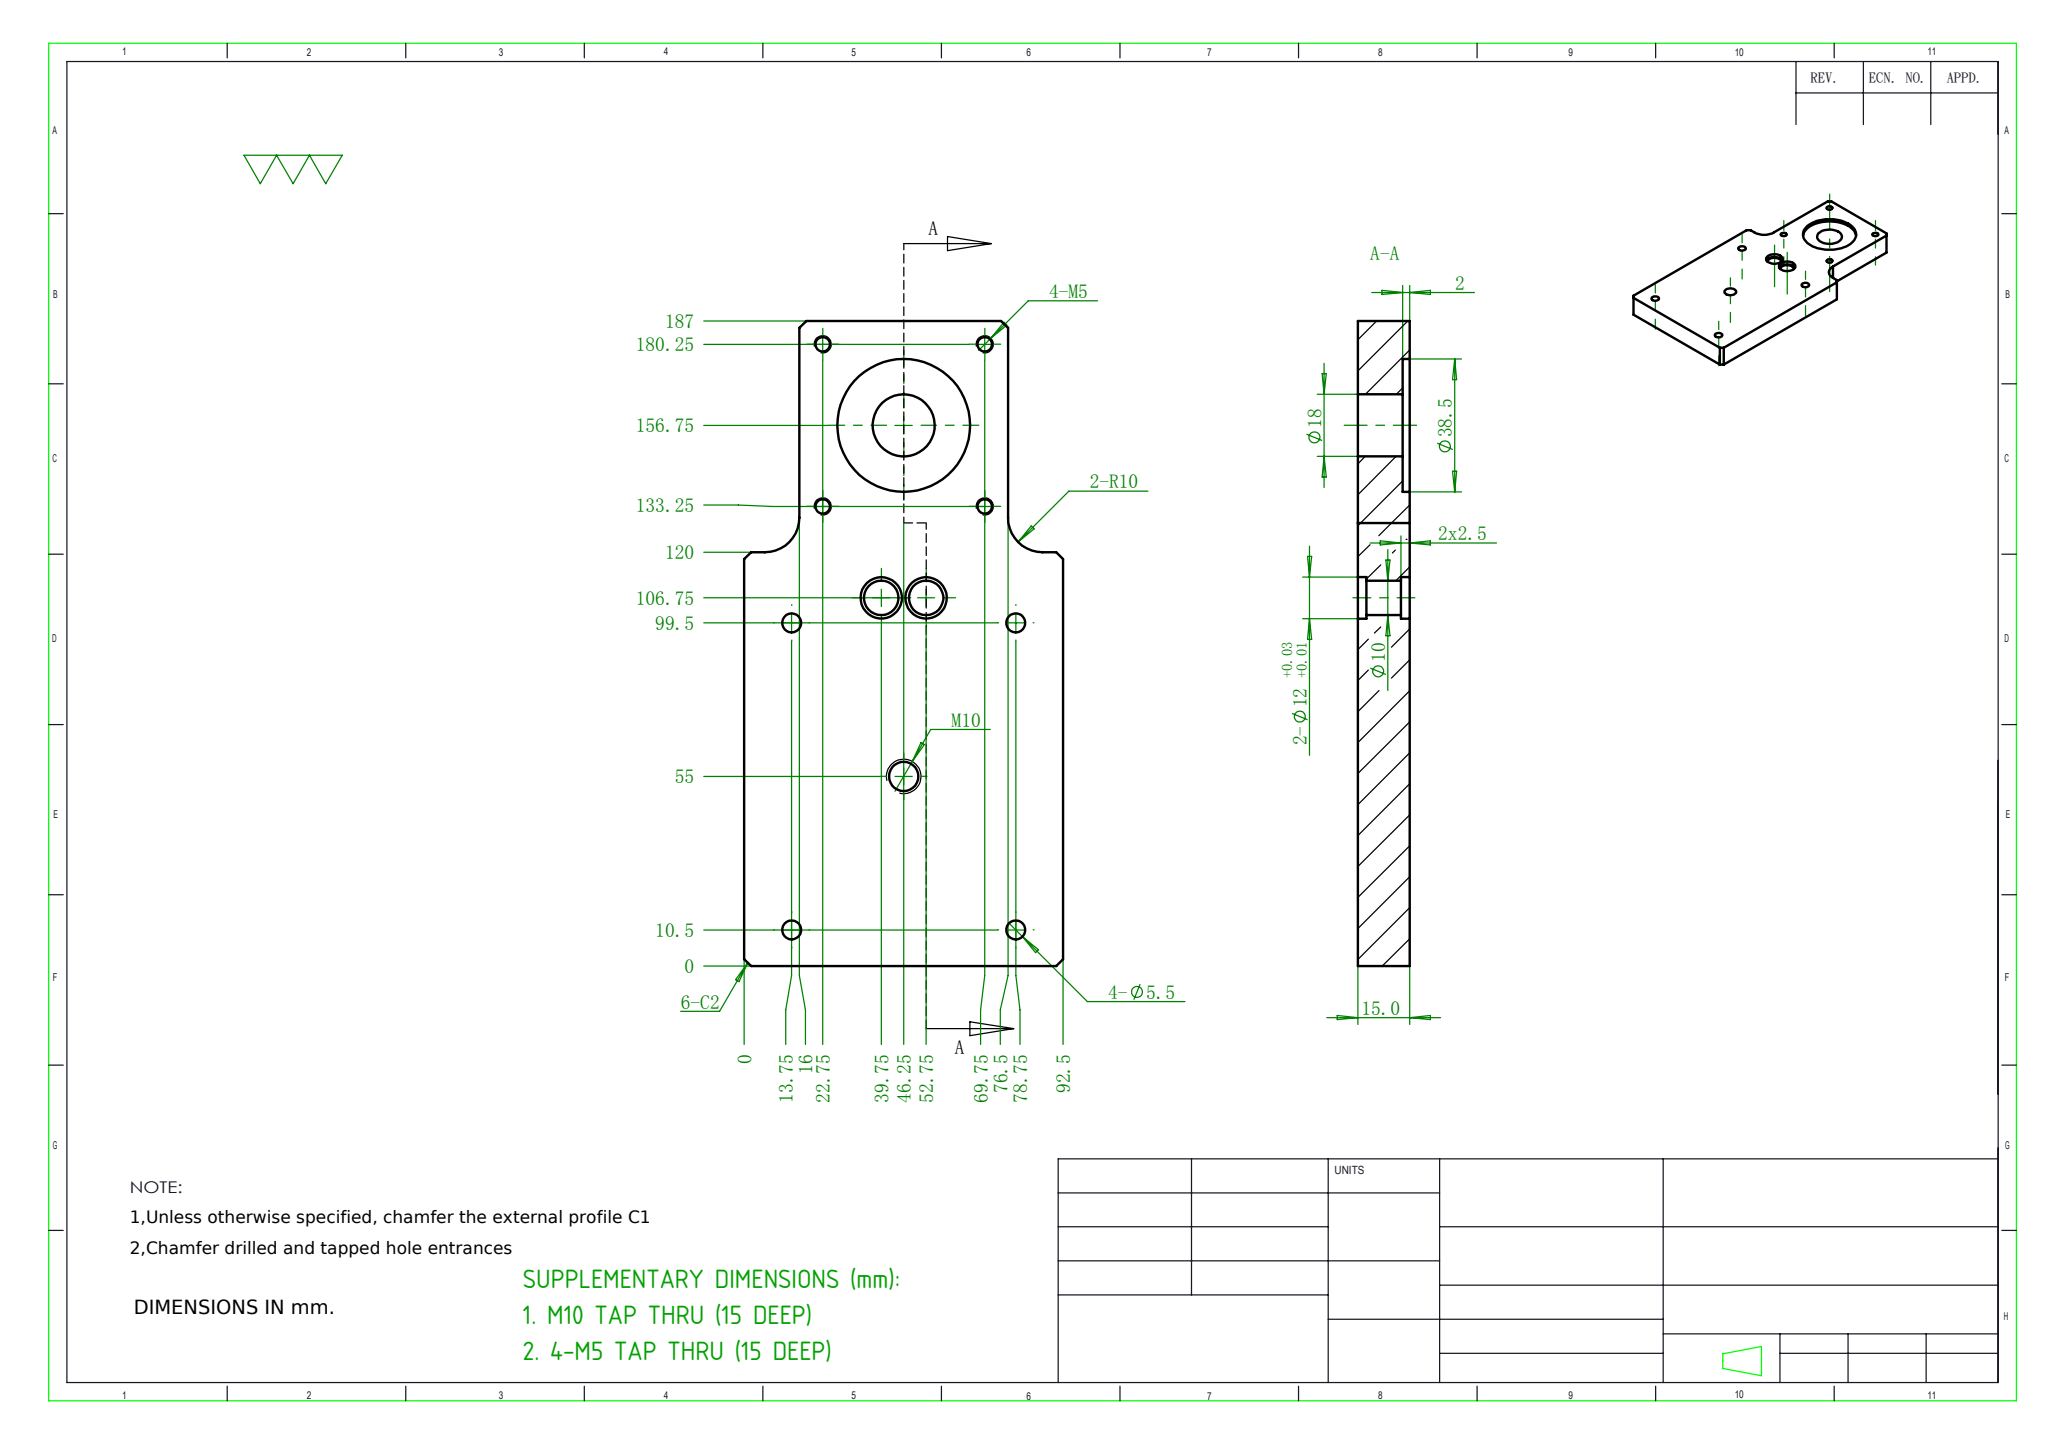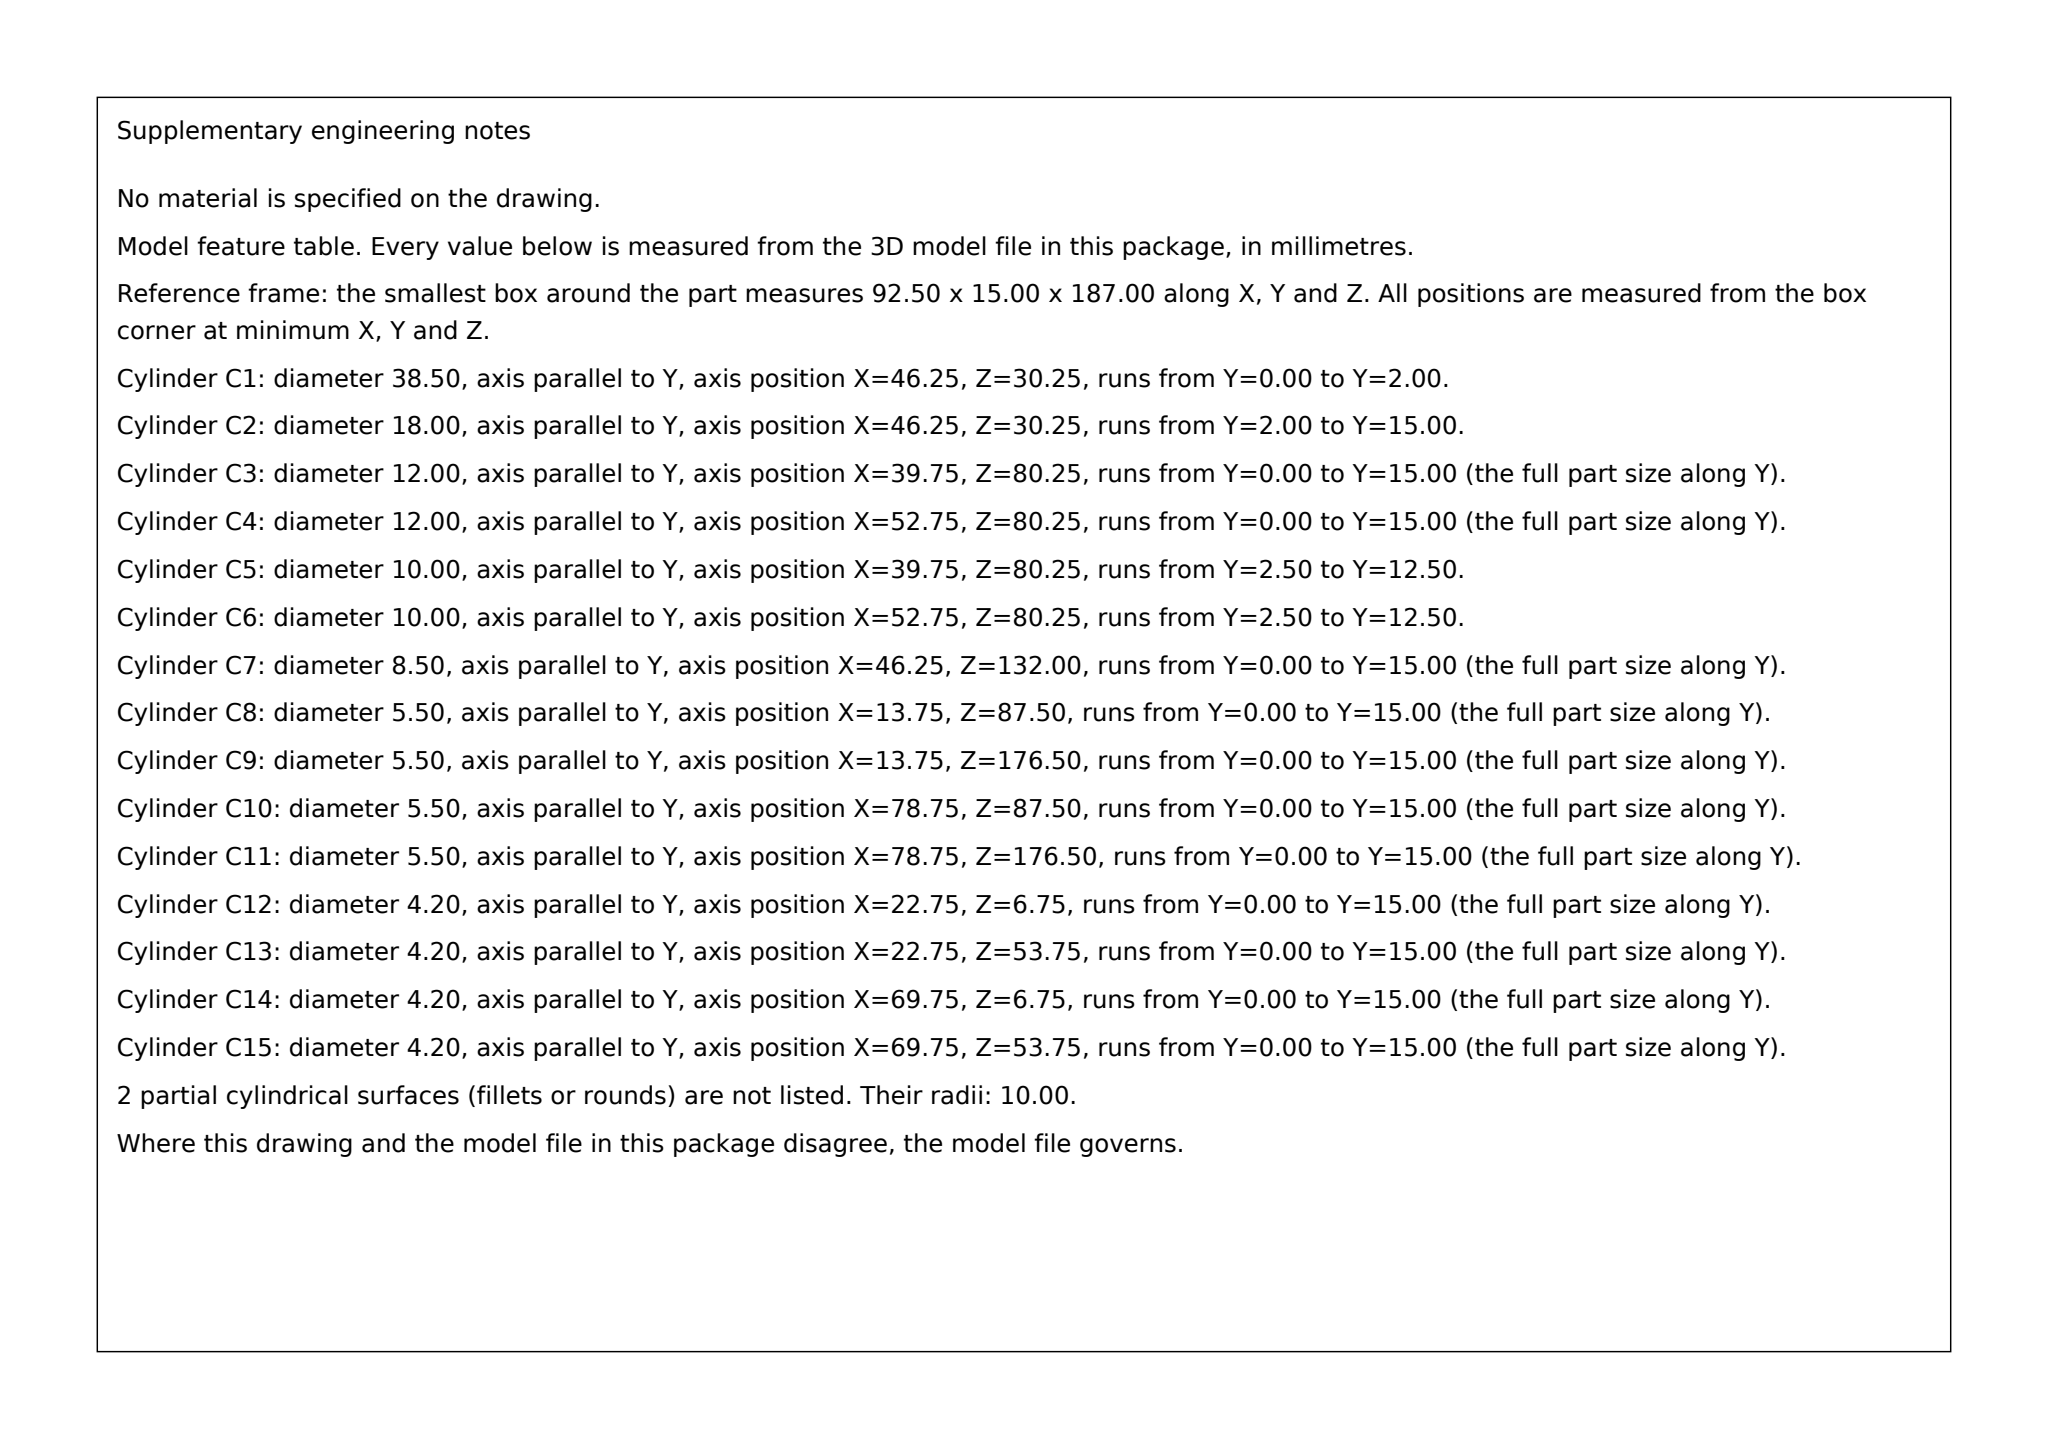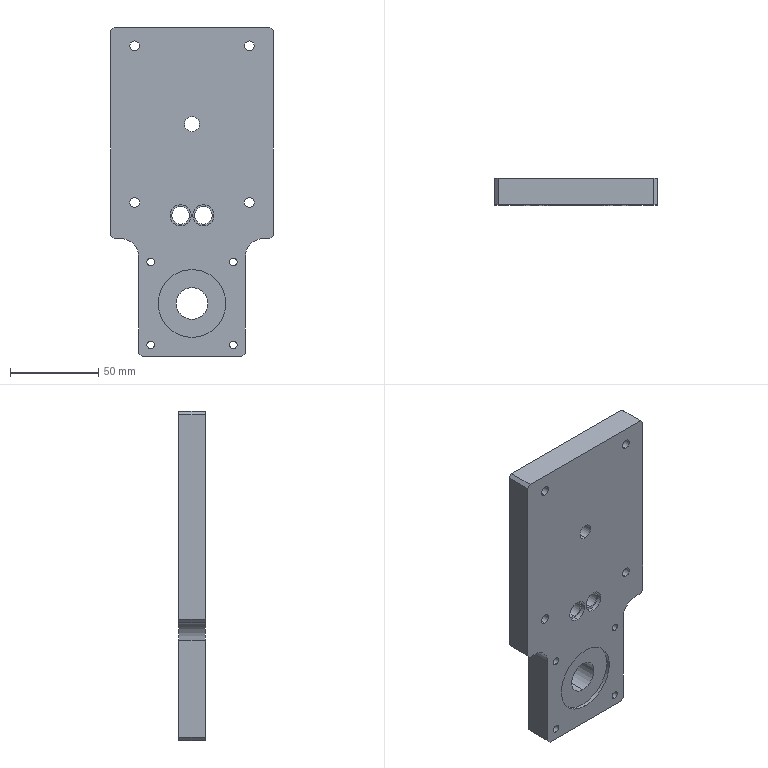Part | SolidWorks | mm | 1 solid | 57 faces | box 92.5 x 15 x 187 mm | volume 216320 mm3 | cylinder 36 | plane 21 | commonest cylinder face diameters 4.2 x8 12 x8 5.5 x8 10 x4 38.5 x2 8.5 x2 18 x2 20 x2
build123d program:
from build123d import *

# Parameters (mm, degrees)
BOSS_EXTRUDE1_DEPTH        = 15
F_5_5_5_5_DIAMETER_HOLE1_D = 5.5
F_6_2_6_2_DIAMETER_HOLE1_D = 10
F_13_0_13_DIAMETER_HOLE1_D = 18
SKETCH11_R                 = 6
CUT_EXTRUDE1_DEPTH         = 2.5
CUT_EXTRUDE2_START         = -2.5
SKETCH12_R                 = 6
CUT_EXTRUDE2_DEPTH         = 2.5
FILLET1_R                  = 10
SKETCH13_W                 = 92.5
SKETCH13_H                 = 15
CUT_EXTRUDE3_DEPTH         = 10
CHAMFER1_SIZE              = 2
M5_TAPPED_HOLE1_D          = 4.2
M10_TAPPED_HOLE1_D         = 8.5
SKETCH18_R                 = 19.25
CUT_EXTRUDE4_DEPTH         = 2


with BuildPart() as part:
    # Sketch1 → Boss-Extrude1 (new body)
    with BuildSketch(Plane(origin=(0, 0, 0), x_dir=(1, 0, 0), z_dir=(0, 1, 0))):
        Polygon((-46.25, 0), (-46.25, 130), (-30.25, 130), (-30.25, 197), (30.25, 197), (30.25, 130), (46.25, 130), (46.25, 0), align=None)
    extrude(amount=BOSS_EXTRUDE1_DEPTH)

    # 5.5 _5.5_ Diameter Hole1 (through all)
    with Locations(Plane(origin=(0, 15, 0), x_dir=(1, 0, 0), z_dir=(0, 1, 0))):
        with Locations((32.5, 20.5), (32.5, 109.5), (-32.5, 109.5), (-32.5, 20.5)):
            Hole(F_5_5_5_5_DIAMETER_HOLE1_D / 2)

    # 6.2 _6.2_ Diameter Hole1 (through all)
    with Locations(Plane(origin=(0, 15, 0), x_dir=(1, 0, 0), z_dir=(0, 1, 0))):
        with Locations((-6.5, 116.75), (6.5, 116.75)):
            Hole(F_6_2_6_2_DIAMETER_HOLE1_D / 2)

    # 13.0 _13_ Diameter Hole1 (through all)
    with Locations(Plane(origin=(0, 15, 0), x_dir=(1, 0, 0), z_dir=(0, 1, 0))):
        with Locations((0, 166.75)):
            Hole(F_13_0_13_DIAMETER_HOLE1_D / 2)

    # Sketch11 → Cut-Extrude1 (cut)
    with BuildSketch(Plane(origin=(0, 15, 0), x_dir=(1, 0, 0), z_dir=(0, 1, 0))):
        with Locations(Location((-6.5, 116.75, 0), (0, 0, 270))):
            Circle(SKETCH11_R)
        with Locations(Location((6.5, 116.75, 0), (0, 0, 270))):
            Circle(SKETCH11_R)
    extrude(amount=-CUT_EXTRUDE1_DEPTH, mode=Mode.SUBTRACT)

    # Sketch12 → Cut-Extrude2 (cut)
    with BuildSketch(Plane.XZ.offset(CUT_EXTRUDE2_START)):
        with Locations(Location((6.5, -116.75, 0), (0, 0, 90))):
            Circle(SKETCH12_R)
        with Locations(Location((-6.5, -116.75, 0), (0, 0, 90))):
            Circle(SKETCH12_R)
    extrude(amount=CUT_EXTRUDE2_DEPTH, mode=Mode.SUBTRACT)

    # Fillet1
    fillet1_edges = [part.edges().sort_by_distance(p)[0] for p in [
        (-30.25, 7.5, -130),
        (30.25, 7.5, -130),
    ]]
    fillet(fillet1_edges, radius=FILLET1_R)

    # Sketch13 → Cut-Extrude3 (cut)
    with BuildSketch(Plane.XY):
        with Locations((0, 7.5)):
            Rectangle(SKETCH13_W, SKETCH13_H)
    extrude(amount=-CUT_EXTRUDE3_DEPTH, mode=Mode.SUBTRACT)

    # Chamfer1
    chamfer1_edges = [part.edges().sort_by_distance(p)[0] for p in [
        (-46.25, 7.5, -10),
        (46.25, 7.5, -10),
        (-46.25, 7.5, -130),
        (-30.25, 7.5, -197),
        (30.25, 7.5, -197),
        (46.25, 7.5, -130),
    ]]
    chamfer(chamfer1_edges, length=CHAMFER1_SIZE)

    # M5 Tapped Hole1 (through all)
    with Locations(Plane(origin=(0, 0, 0), x_dir=(-1, 0, 0), z_dir=(0, -1, 0))):
        with Locations((23.5, 143.25), (-23.5, 143.25), (-23.5, 190.25), (23.5, 190.25)):
            Hole(M5_TAPPED_HOLE1_D / 2)

    # M10 Tapped Hole1 (through all)
    with Locations(Plane(origin=(0, 15, 0), x_dir=(1, 0, 0), z_dir=(0, 1, 0))):
        with Locations((0, 65)):
            Hole(M10_TAPPED_HOLE1_D / 2)

    # Sketch18 → Cut-Extrude4 (cut)
    with BuildSketch(Plane.XZ):
        with Locations(Location((0, -166.75, 0), (0, 0, 270))):
            Circle(SKETCH18_R)
    extrude(amount=-CUT_EXTRUDE4_DEPTH, mode=Mode.SUBTRACT)


solid = part.part